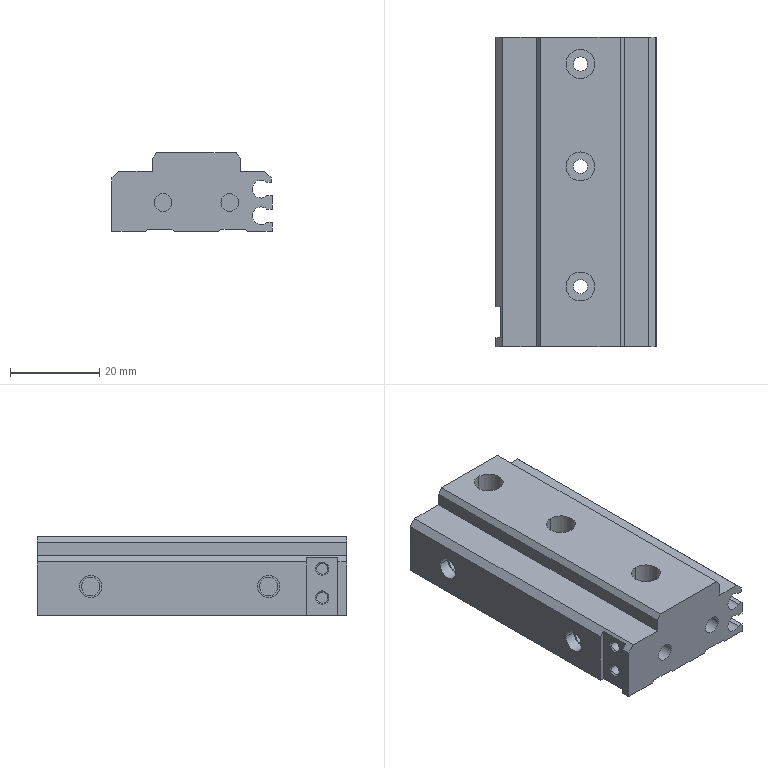Component | SolidWorks | MXQ8-30B-M9N_0_0_MXQ8-30B-M9N_0_0-2_MXQ8-30B-M9N_0_0_1_26-1 | 1 solid | 135 faces | volume 31460 mm3 | cylinder 59 | plane 58 | cone 18 | commonest cylinder face diameters 2.459 x12 4 x8 6.5 x6 3.2 x6 3.242 x6 3 x5 4.134 x4 5 x4